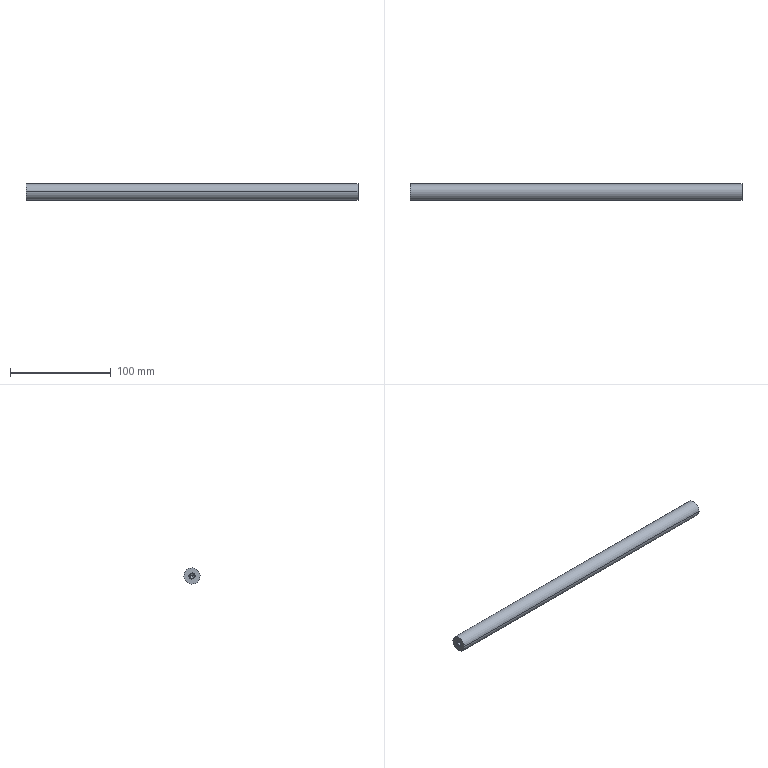Component | SolidWorks | DoubleFilmTransport-1_GuideRod-2 | 1 solid | 16 faces | box 330 x 16 x 16 mm | volume 65501 mm3 | cone 8 | cylinder 6 | plane 2 | commonest cylinder face diameters 5 x4 16 x2
build123d program:
from build123d import *


with BuildPart() as part:
    # Sketch1 → Revolve1 (revolve)
    with BuildSketch(Plane.XZ, mode=Mode.PRIVATE) as revolve1_sk:
        Polygon((2.5, 144), (0, 142.498), (0, -142.498), (2.5, -144), (2.5, -164.475), (3.025, -165), (8, -165), (8, 165), (3.025, 165), (2.5, 164.475), align=None)
    revolve(revolve1_sk.sketch.rotate(Axis((0, 0, 165), (0, 0, -1)), 180), axis=Axis((0, 0, 165), (0, 0, -1)))


solid = part.part

# Placed as in the assembly
solid = solid.moved(Location((-300.059, 45.373, 13.5), (0, 90, 0)))
STEP:
#1=COLOUR_RGB('',0.7922,0.8196,0.9333);
#2=FILL_AREA_STYLE_COLOUR('',#1);
#3=FILL_AREA_STYLE('',(#2));
#4=SURFACE_STYLE_FILL_AREA(#3);
#5=SURFACE_SIDE_STYLE('',(#4));
#6=SURFACE_STYLE_USAGE(.BOTH.,#5);
#7=PRESENTATION_STYLE_ASSIGNMENT((#6));
#8=CARTESIAN_POINT('',(-5.338,1.885,0.5242));
#9=VERTEX_POINT('',#8);
#10=CARTESIAN_POINT('',(-5.338,1.688,0.5388));
#11=VERTEX_POINT('',#10);
#12=CARTESIAN_POINT('',(-5.338,1.786,0.5315));
#13=DIRECTION('',(-1.,-0.,-0.));
#14=DIRECTION('',(0.,-0.9973,0.0739));
#15=AXIS2_PLACEMENT_3D('',#12,#13,#14);
#16=CIRCLE('',#15,0.09843);
#17=EDGE_CURVE('',#9,#11,#16,.T.);
#18=ORIENTED_EDGE('',*,*,#17,.T.);
#19=CARTESIAN_POINT('',(-5.317,1.668,0.5403));
#20=VERTEX_POINT('',#19);
#21=CARTESIAN_POINT('',(-5.317,1.668,0.5403));
#22=DIRECTION('',(0.7071,-0.7052,0.05225));
#23=VECTOR('',#22,39.37);
#24=LINE('',#21,#23);
#25=EDGE_CURVE('',#11,#20,#24,.T.);
#26=ORIENTED_EDGE('',*,*,#25,.T.);
#27=CARTESIAN_POINT('',(-5.317,1.905,0.5227));
#28=VERTEX_POINT('',#27);
#29=CARTESIAN_POINT('',(-5.317,1.786,0.5315));
#30=DIRECTION('',(-1.,-0.,-0.));
#31=DIRECTION('',(0.,-0.9973,0.0739));
#32=AXIS2_PLACEMENT_3D('',#29,#30,#31);
#33=CIRCLE('',#32,0.1191);
#34=EDGE_CURVE('',#28,#20,#33,.T.);
#35=ORIENTED_EDGE('',*,*,#34,.F.);
#36=CARTESIAN_POINT('',(-5.317,1.905,0.5227));
#37=DIRECTION('',(0.7071,0.7052,-0.05225));
#38=VECTOR('',#37,39.37);
#39=LINE('',#36,#38);
#40=EDGE_CURVE('',#9,#28,#39,.T.);
#41=ORIENTED_EDGE('',*,*,#40,.F.);
#42=EDGE_LOOP('',(#18,#26,#35,#41));
#43=FACE_OUTER_BOUND('',#42,.T.);
#44=CARTESIAN_POINT('',(-5.317,1.786,0.5315));
#45=DIRECTION('',(1.,0.,0.));
#46=DIRECTION('',(0.,0.9973,-0.0739));
#47=AXIS2_PLACEMENT_3D('',#44,#45,#46);
#48=CONICAL_SURFACE('',#47,0.1191,0.7854);
#49=ADVANCED_FACE('',(#43),#48,.F.);
#50=CARTESIAN_POINT('',(-5.317,1.472,0.5548));
#51=VERTEX_POINT('',#50);
#52=CARTESIAN_POINT('',(-5.317,2.1,0.5082));
#53=VERTEX_POINT('',#52);
#54=CARTESIAN_POINT('',(-5.317,1.786,0.5315));
#55=DIRECTION('',(-1.,-0.,-0.));
#56=DIRECTION('',(0.,-0.9973,0.0739));
#57=AXIS2_PLACEMENT_3D('',#54,#55,#56);
#58=CIRCLE('',#57,0.315);
#59=EDGE_CURVE('',#51,#53,#58,.T.);
#60=ORIENTED_EDGE('',*,*,#59,.T.);
#61=CARTESIAN_POINT('',(-18.309,2.1,0.5082));
#62=VERTEX_POINT('',#61);
#63=CARTESIAN_POINT('',(-5.317,2.1,0.5082));
#64=DIRECTION('',(-1.,-0.,-0.));
#65=VECTOR('',#64,39.37);
#66=LINE('',#63,#65);
#67=EDGE_CURVE('',#53,#62,#66,.T.);
#68=ORIENTED_EDGE('',*,*,#67,.T.);
#69=CARTESIAN_POINT('',(-18.309,1.472,0.5548));
#70=VERTEX_POINT('',#69);
#71=CARTESIAN_POINT('',(-18.309,1.786,0.5315));
#72=DIRECTION('',(-1.,-0.,-0.));
#73=DIRECTION('',(0.,-0.9973,0.0739));
#74=AXIS2_PLACEMENT_3D('',#71,#72,#73);
#75=CIRCLE('',#74,0.315);
#76=EDGE_CURVE('',#70,#62,#75,.T.);
#77=ORIENTED_EDGE('',*,*,#76,.F.);
#78=CARTESIAN_POINT('',(-5.317,1.472,0.5548));
#79=DIRECTION('',(-1.,-0.,-0.));
#80=VECTOR('',#79,39.37);
#81=LINE('',#78,#80);
#82=EDGE_CURVE('',#51,#70,#81,.T.);
#83=ORIENTED_EDGE('',*,*,#82,.F.);
#84=EDGE_LOOP('',(#60,#68,#77,#83));
#85=FACE_OUTER_BOUND('',#84,.T.);
#86=CARTESIAN_POINT('',(-5.317,1.786,0.5315));
#87=DIRECTION('',(-1.,-0.,-0.));
#88=DIRECTION('',(0.,-0.9973,0.0739));
#89=AXIS2_PLACEMENT_3D('',#86,#87,#88);
#90=CYLINDRICAL_SURFACE('',#89,0.315);
#91=ADVANCED_FACE('',(#85),#90,.T.);
#92=CARTESIAN_POINT('',(-18.289,1.885,0.5242));
#93=VERTEX_POINT('',#92);
#94=CARTESIAN_POINT('',(-18.289,1.688,0.5388));
#95=VERTEX_POINT('',#94);
#96=CARTESIAN_POINT('',(-18.289,1.786,0.5315));
#97=DIRECTION('',(-1.,-0.,-0.));
#98=DIRECTION('',(0.,-0.9973,0.0739));
#99=AXIS2_PLACEMENT_3D('',#96,#97,#98);
#100=CIRCLE('',#99,0.09843);
#101=EDGE_CURVE('',#93,#95,#100,.T.);
#102=ORIENTED_EDGE('',*,*,#101,.F.);
#103=CARTESIAN_POINT('',(-18.309,1.905,0.5227));
#104=VERTEX_POINT('',#103);
#105=CARTESIAN_POINT('',(-18.289,1.885,0.5242));
#106=DIRECTION('',(-0.7071,0.7052,-0.05225));
#107=VECTOR('',#106,39.37);
#108=LINE('',#105,#107);
#109=EDGE_CURVE('',#93,#104,#108,.T.);
#110=ORIENTED_EDGE('',*,*,#109,.T.);
#111=CARTESIAN_POINT('',(-18.309,1.668,0.5403));
#112=VERTEX_POINT('',#111);
#113=CARTESIAN_POINT('',(-18.309,1.786,0.5315));
#114=DIRECTION('',(-1.,-0.,-0.));
#115=DIRECTION('',(0.,-0.9973,0.0739));
#116=AXIS2_PLACEMENT_3D('',#113,#114,#115);
#117=CIRCLE('',#116,0.1191);
#118=EDGE_CURVE('',#104,#112,#117,.T.);
#119=ORIENTED_EDGE('',*,*,#118,.T.);
#120=CARTESIAN_POINT('',(-18.289,1.688,0.5388));
#121=DIRECTION('',(-0.7071,-0.7052,0.05225));
#122=VECTOR('',#121,39.37);
#123=LINE('',#120,#122);
#124=EDGE_CURVE('',#95,#112,#123,.T.);
#125=ORIENTED_EDGE('',*,*,#124,.F.);
#126=EDGE_LOOP('',(#102,#110,#119,#125));
#127=FACE_OUTER_BOUND('',#126,.T.);
#128=CARTESIAN_POINT('',(-18.289,1.786,0.5315));
#129=DIRECTION('',(-1.,-0.,-0.));
#130=DIRECTION('',(0.,-0.9973,0.0739));
#131=AXIS2_PLACEMENT_3D('',#128,#129,#130);
#132=CONICAL_SURFACE('',#131,0.09843,0.7854);
#133=ADVANCED_FACE('',(#127),#132,.F.);
#134=CARTESIAN_POINT('',(-17.483,1.885,0.5242));
#135=VERTEX_POINT('',#134);
#136=CARTESIAN_POINT('',(-17.483,1.688,0.5388));
#137=VERTEX_POINT('',#136);
#138=CARTESIAN_POINT('',(-17.483,1.786,0.5315));
#139=DIRECTION('',(-1.,-0.,-0.));
#140=DIRECTION('',(0.,-0.9973,0.0739));
#141=AXIS2_PLACEMENT_3D('',#138,#139,#140);
#142=CIRCLE('',#141,0.09843);
#143=EDGE_CURVE('',#135,#137,#142,.T.);
#144=ORIENTED_EDGE('',*,*,#143,.F.);
#145=CARTESIAN_POINT('',(-5.317,1.885,0.5242));
#146=DIRECTION('',(-1.,-0.,-0.));
#147=VECTOR('',#146,39.37);
#148=LINE('',#145,#147);
#149=EDGE_CURVE('',#135,#93,#148,.T.);
#150=ORIENTED_EDGE('',*,*,#149,.T.);
#151=ORIENTED_EDGE('',*,*,#101,.T.);
#152=CARTESIAN_POINT('',(-5.317,1.688,0.5388));
#153=DIRECTION('',(-1.,-0.,-0.));
#154=VECTOR('',#153,39.37);
#155=LINE('',#152,#154);
#156=EDGE_CURVE('',#137,#95,#155,.T.);
#157=ORIENTED_EDGE('',*,*,#156,.F.);
#158=EDGE_LOOP('',(#144,#150,#151,#157));
#159=FACE_OUTER_BOUND('',#158,.T.);
#160=CARTESIAN_POINT('',(-5.317,1.786,0.5315));
#161=DIRECTION('',(-1.,-0.,-0.));
#162=DIRECTION('',(0.,-0.9973,0.0739));
#163=AXIS2_PLACEMENT_3D('',#160,#161,#162);
#164=CYLINDRICAL_SURFACE('',#163,0.09843);
#165=ADVANCED_FACE('',(#159),#164,.F.);
#166=CARTESIAN_POINT('',(-17.424,1.786,0.5315));
#167=VERTEX_POINT('',#166);
#168=CARTESIAN_POINT('',(-17.424,1.786,0.5315));
#169=DIRECTION('',(-0.515,-0.8548,0.06334));
#170=VECTOR('',#169,39.37);
#171=LINE('',#168,#170);
#172=EDGE_CURVE('',#167,#137,#171,.T.);
#173=ORIENTED_EDGE('',*,*,#172,.F.);
#174=CARTESIAN_POINT('',(-17.424,1.786,0.5315));
#175=DIRECTION('',(-0.515,0.8548,-0.06334));
#176=VECTOR('',#175,39.37);
#177=LINE('',#174,#176);
#178=EDGE_CURVE('',#167,#135,#177,.T.);
#179=ORIENTED_EDGE('',*,*,#178,.T.);
#180=ORIENTED_EDGE('',*,*,#143,.T.);
#181=EDGE_LOOP('',(#173,#179,#180));
#182=FACE_OUTER_BOUND('',#181,.T.);
#183=CARTESIAN_POINT('',(-56.794,1.786,0.5315));
#184=DIRECTION('',(-1.,-0.,-0.));
#185=DIRECTION('',(0.,-0.9973,0.0739));
#186=AXIS2_PLACEMENT_3D('',#183,#184,#185);
#187=CONICAL_SURFACE('',#186,65.523,1.03);
#188=ADVANCED_FACE('',(#182),#187,.F.);
#189=CARTESIAN_POINT('',(-6.203,1.786,0.5315));
#190=VERTEX_POINT('',#189);
#191=CARTESIAN_POINT('',(-6.144,1.885,0.5242));
#192=VERTEX_POINT('',#191);
#193=CARTESIAN_POINT('',(-6.144,1.885,0.5242));
#194=DIRECTION('',(0.515,0.8548,-0.06334));
#195=VECTOR('',#194,39.37);
#196=LINE('',#193,#195);
#197=EDGE_CURVE('',#190,#192,#196,.T.);
#198=ORIENTED_EDGE('',*,*,#197,.F.);
#199=CARTESIAN_POINT('',(-6.144,1.688,0.5388));
#200=VERTEX_POINT('',#199);
#201=CARTESIAN_POINT('',(-6.144,1.688,0.5388));
#202=DIRECTION('',(0.515,-0.8548,0.06334));
#203=VECTOR('',#202,39.37);
#204=LINE('',#201,#203);
#205=EDGE_CURVE('',#190,#200,#204,.T.);
#206=ORIENTED_EDGE('',*,*,#205,.T.);
#207=CARTESIAN_POINT('',(-6.144,1.786,0.5315));
#208=DIRECTION('',(-1.,-0.,-0.));
#209=DIRECTION('',(0.,-0.9973,0.0739));
#210=AXIS2_PLACEMENT_3D('',#207,#208,#209);
#211=CIRCLE('',#210,0.09843);
#212=EDGE_CURVE('',#192,#200,#211,.T.);
#213=ORIENTED_EDGE('',*,*,#212,.F.);
#214=EDGE_LOOP('',(#198,#206,#213));
#215=FACE_OUTER_BOUND('',#214,.T.);
#216=CARTESIAN_POINT('',(-6.144,1.786,0.5315));
#217=DIRECTION('',(1.,0.,0.));
#218=DIRECTION('',(0.,0.9973,-0.0739));
#219=AXIS2_PLACEMENT_3D('',#216,#217,#218);
#220=CONICAL_SURFACE('',#219,0.09843,1.03);
#221=ADVANCED_FACE('',(#215),#220,.F.);
#222=ORIENTED_EDGE('',*,*,#17,.F.);
#223=CARTESIAN_POINT('',(-5.317,1.885,0.5242));
#224=DIRECTION('',(-1.,-0.,-0.));
#225=VECTOR('',#224,39.37);
#226=LINE('',#223,#225);
#227=EDGE_CURVE('',#9,#192,#226,.T.);
#228=ORIENTED_EDGE('',*,*,#227,.T.);
#229=ORIENTED_EDGE('',*,*,#212,.T.);
#230=CARTESIAN_POINT('',(-5.317,1.688,0.5388));
#231=DIRECTION('',(-1.,-0.,-0.));
#232=VECTOR('',#231,39.37);
#233=LINE('',#230,#232);
#234=EDGE_CURVE('',#11,#200,#233,.T.);
#235=ORIENTED_EDGE('',*,*,#234,.F.);
#236=EDGE_LOOP('',(#222,#228,#229,#235));
#237=FACE_OUTER_BOUND('',#236,.T.);
#238=CARTESIAN_POINT('',(-5.317,1.786,0.5315));
#239=DIRECTION('',(-1.,-0.,-0.));
#240=DIRECTION('',(0.,-0.9973,0.0739));
#241=AXIS2_PLACEMENT_3D('',#238,#239,#240);
#242=CYLINDRICAL_SURFACE('',#241,0.09843);
#243=ADVANCED_FACE('',(#237),#242,.F.);
#244=ORIENTED_EDGE('',*,*,#227,.F.);
#245=CARTESIAN_POINT('',(-5.338,1.786,0.5315));
#246=DIRECTION('',(-1.,-0.,-0.));
#247=DIRECTION('',(0.,-0.9973,0.0739));
#248=AXIS2_PLACEMENT_3D('',#245,#246,#247);
#249=CIRCLE('',#248,0.09843);
#250=EDGE_CURVE('',#11,#9,#249,.T.);
#251=ORIENTED_EDGE('',*,*,#250,.F.);
#252=ORIENTED_EDGE('',*,*,#234,.T.);
#253=CARTESIAN_POINT('',(-6.144,1.786,0.5315));
#254=DIRECTION('',(-1.,-0.,-0.));
#255=DIRECTION('',(0.,-0.9973,0.0739));
#256=AXIS2_PLACEMENT_3D('',#253,#254,#255);
#257=CIRCLE('',#256,0.09843);
#258=EDGE_CURVE('',#200,#192,#257,.T.);
#259=ORIENTED_EDGE('',*,*,#258,.T.);
#260=EDGE_LOOP('',(#244,#251,#252,#259));
#261=FACE_OUTER_BOUND('',#260,.T.);
#262=CARTESIAN_POINT('',(-5.317,1.786,0.5315));
#263=DIRECTION('',(-1.,-0.,-0.));
#264=DIRECTION('',(0.,-0.9973,0.0739));
#265=AXIS2_PLACEMENT_3D('',#262,#263,#264);
#266=CYLINDRICAL_SURFACE('',#265,0.09843);
#267=ADVANCED_FACE('',(#261),#266,.F.);
#268=ORIENTED_EDGE('',*,*,#205,.F.);
#269=ORIENTED_EDGE('',*,*,#197,.T.);
#270=ORIENTED_EDGE('',*,*,#258,.F.);
#271=EDGE_LOOP('',(#268,#269,#270));
#272=FACE_OUTER_BOUND('',#271,.T.);
#273=CARTESIAN_POINT('',(-6.144,1.786,0.5315));
#274=DIRECTION('',(1.,0.,0.));
#275=DIRECTION('',(0.,0.9973,-0.0739));
#276=AXIS2_PLACEMENT_3D('',#273,#274,#275);
#277=CONICAL_SURFACE('',#276,0.09843,1.03);
#278=ADVANCED_FACE('',(#272),#277,.F.);
#279=ORIENTED_EDGE('',*,*,#178,.F.);
#280=ORIENTED_EDGE('',*,*,#172,.T.);
#281=CARTESIAN_POINT('',(-17.483,1.786,0.5315));
#282=DIRECTION('',(-1.,-0.,-0.));
#283=DIRECTION('',(0.,-0.9973,0.0739));
#284=AXIS2_PLACEMENT_3D('',#281,#282,#283);
#285=CIRCLE('',#284,0.09843);
#286=EDGE_CURVE('',#137,#135,#285,.T.);
#287=ORIENTED_EDGE('',*,*,#286,.T.);
#288=EDGE_LOOP('',(#279,#280,#287));
#289=FACE_OUTER_BOUND('',#288,.T.);
#290=CARTESIAN_POINT('',(-56.794,1.786,0.5315));
#291=DIRECTION('',(-1.,-0.,-0.));
#292=DIRECTION('',(0.,-0.9973,0.0739));
#293=AXIS2_PLACEMENT_3D('',#290,#291,#292);
#294=CONICAL_SURFACE('',#293,65.523,1.03);
#295=ADVANCED_FACE('',(#289),#294,.F.);
#296=ORIENTED_EDGE('',*,*,#149,.F.);
#297=ORIENTED_EDGE('',*,*,#286,.F.);
#298=ORIENTED_EDGE('',*,*,#156,.T.);
#299=CARTESIAN_POINT('',(-18.289,1.786,0.5315));
#300=DIRECTION('',(-1.,-0.,-0.));
#301=DIRECTION('',(0.,-0.9973,0.0739));
#302=AXIS2_PLACEMENT_3D('',#299,#300,#301);
#303=CIRCLE('',#302,0.09843);
#304=EDGE_CURVE('',#95,#93,#303,.T.);
#305=ORIENTED_EDGE('',*,*,#304,.T.);
#306=EDGE_LOOP('',(#296,#297,#298,#305));
#307=FACE_OUTER_BOUND('',#306,.T.);
#308=CARTESIAN_POINT('',(-5.317,1.786,0.5315));
#309=DIRECTION('',(-1.,-0.,-0.));
#310=DIRECTION('',(0.,-0.9973,0.0739));
#311=AXIS2_PLACEMENT_3D('',#308,#309,#310);
#312=CYLINDRICAL_SURFACE('',#311,0.09843);
#313=ADVANCED_FACE('',(#307),#312,.F.);
#314=ORIENTED_EDGE('',*,*,#109,.F.);
#315=ORIENTED_EDGE('',*,*,#304,.F.);
#316=ORIENTED_EDGE('',*,*,#124,.T.);
#317=CARTESIAN_POINT('',(-18.309,1.786,0.5315));
#318=DIRECTION('',(-1.,-0.,-0.));
#319=DIRECTION('',(0.,-0.9973,0.0739));
#320=AXIS2_PLACEMENT_3D('',#317,#318,#319);
#321=CIRCLE('',#320,0.1191);
#322=EDGE_CURVE('',#112,#104,#321,.T.);
#323=ORIENTED_EDGE('',*,*,#322,.T.);
#324=EDGE_LOOP('',(#314,#315,#316,#323));
#325=FACE_OUTER_BOUND('',#324,.T.);
#326=CARTESIAN_POINT('',(-18.289,1.786,0.5315));
#327=DIRECTION('',(-1.,-0.,-0.));
#328=DIRECTION('',(0.,-0.9973,0.0739));
#329=AXIS2_PLACEMENT_3D('',#326,#327,#328);
#330=CONICAL_SURFACE('',#329,0.09843,0.7854);
#331=ADVANCED_FACE('',(#325),#330,.F.);
#332=ORIENTED_EDGE('',*,*,#76,.T.);
#333=CARTESIAN_POINT('',(-18.309,1.786,0.5315));
#334=DIRECTION('',(-1.,-0.,-0.));
#335=DIRECTION('',(0.,-0.9973,0.0739));
#336=AXIS2_PLACEMENT_3D('',#333,#334,#335);
#337=CIRCLE('',#336,0.315);
#338=EDGE_CURVE('',#62,#70,#337,.T.);
#339=ORIENTED_EDGE('',*,*,#338,.T.);
#340=EDGE_LOOP('',(#332,#339));
#341=FACE_OUTER_BOUND('',#340,.T.);
#342=ORIENTED_EDGE('',*,*,#322,.F.);
#343=ORIENTED_EDGE('',*,*,#118,.F.);
#344=EDGE_LOOP('',(#342,#343));
#345=FACE_BOUND('',#344,.T.);
#346=CARTESIAN_POINT('',(-18.309,1.905,0.5227));
#347=DIRECTION('',(-1.,-0.,-0.));
#348=DIRECTION('',(0.,-0.9973,0.0739));
#349=AXIS2_PLACEMENT_3D('',#346,#347,#348);
#350=PLANE('',#349);
#351=ADVANCED_FACE('',(#341,#345),#350,.T.);
#352=ORIENTED_EDGE('',*,*,#67,.F.);
#353=CARTESIAN_POINT('',(-5.317,1.786,0.5315));
#354=DIRECTION('',(-1.,-0.,-0.));
#355=DIRECTION('',(0.,-0.9973,0.0739));
#356=AXIS2_PLACEMENT_3D('',#353,#354,#355);
#357=CIRCLE('',#356,0.315);
#358=EDGE_CURVE('',#53,#51,#357,.T.);
#359=ORIENTED_EDGE('',*,*,#358,.T.);
#360=ORIENTED_EDGE('',*,*,#82,.T.);
#361=ORIENTED_EDGE('',*,*,#338,.F.);
#362=EDGE_LOOP('',(#352,#359,#360,#361));
#363=FACE_OUTER_BOUND('',#362,.T.);
#364=CARTESIAN_POINT('',(-5.317,1.786,0.5315));
#365=DIRECTION('',(-1.,-0.,-0.));
#366=DIRECTION('',(0.,-0.9973,0.0739));
#367=AXIS2_PLACEMENT_3D('',#364,#365,#366);
#368=CYLINDRICAL_SURFACE('',#367,0.315);
#369=ADVANCED_FACE('',(#363),#368,.T.);
#370=ORIENTED_EDGE('',*,*,#34,.T.);
#371=CARTESIAN_POINT('',(-5.317,1.786,0.5315));
#372=DIRECTION('',(-1.,-0.,-0.));
#373=DIRECTION('',(0.,-0.9973,0.0739));
#374=AXIS2_PLACEMENT_3D('',#371,#372,#373);
#375=CIRCLE('',#374,0.1191);
#376=EDGE_CURVE('',#20,#28,#375,.T.);
#377=ORIENTED_EDGE('',*,*,#376,.T.);
#378=EDGE_LOOP('',(#370,#377));
#379=FACE_BOUND('',#378,.T.);
#380=ORIENTED_EDGE('',*,*,#59,.F.);
#381=ORIENTED_EDGE('',*,*,#358,.F.);
#382=EDGE_LOOP('',(#380,#381));
#383=FACE_OUTER_BOUND('',#382,.T.);
#384=CARTESIAN_POINT('',(-5.317,2.1,0.5082));
#385=DIRECTION('',(1.,0.,0.));
#386=DIRECTION('',(-0.,0.9973,-0.0739));
#387=AXIS2_PLACEMENT_3D('',#384,#385,#386);
#388=PLANE('',#387);
#389=ADVANCED_FACE('',(#379,#383),#388,.T.);
#390=ORIENTED_EDGE('',*,*,#25,.F.);
#391=ORIENTED_EDGE('',*,*,#250,.T.);
#392=ORIENTED_EDGE('',*,*,#40,.T.);
#393=ORIENTED_EDGE('',*,*,#376,.F.);
#394=EDGE_LOOP('',(#390,#391,#392,#393));
#395=FACE_OUTER_BOUND('',#394,.T.);
#396=CARTESIAN_POINT('',(-5.317,1.786,0.5315));
#397=DIRECTION('',(1.,0.,0.));
#398=DIRECTION('',(0.,0.9973,-0.0739));
#399=AXIS2_PLACEMENT_3D('',#396,#397,#398);
#400=CONICAL_SURFACE('',#399,0.1191,0.7854);
#401=ADVANCED_FACE('',(#395),#400,.F.);
#402=CLOSED_SHELL('',(#49,#91,#133,#165,#188,#221,#243,#267,#278,#295,#313,#331,#351,#369,#389,#401));
#403=MANIFOLD_SOLID_BREP('',#402);
#404=STYLED_ITEM('',(#7),#403);
#405=(LENGTH_UNIT()NAMED_UNIT(*)SI_UNIT($,.METRE.));
#406=LENGTH_MEASURE_WITH_UNIT(LENGTH_MEASURE(0.0254),#405);
#407=DIMENSIONAL_EXPONENTS(1.,0.,0.,0.,0.,0.,0.);
#408=(CONVERSION_BASED_UNIT('',#406)LENGTH_UNIT()NAMED_UNIT(#407));
#409=UNCERTAINTY_MEASURE_WITH_UNIT(LENGTH_MEASURE(0.00001),#408,'','');
#410=(NAMED_UNIT(*)PLANE_ANGLE_UNIT()SI_UNIT($,.RADIAN.));
#411=(NAMED_UNIT(*)SI_UNIT($,.STERADIAN.)SOLID_ANGLE_UNIT());
#412=(GEOMETRIC_REPRESENTATION_CONTEXT(3)GLOBAL_UNCERTAINTY_ASSIGNED_CONTEXT((#409))GLOBAL_UNIT_ASSIGNED_CONTEXT((#408,#410,#411))REPRESENTATION_CONTEXT('',''));
#413=MECHANICAL_DESIGN_GEOMETRIC_PRESENTATION_REPRESENTATION('',(#404),#412);
#414=CARTESIAN_POINT('',(0.,0.,0.));
#415=DIRECTION('',(0.,0.,1.));
#416=DIRECTION('',(1.,0.,0.));
#417=AXIS2_PLACEMENT_3D('',#414,#415,#416);
#418=(LENGTH_UNIT()NAMED_UNIT(*)SI_UNIT($,.METRE.));
#419=LENGTH_MEASURE_WITH_UNIT(LENGTH_MEASURE(0.0254),#418);
#420=DIMENSIONAL_EXPONENTS(1.,0.,0.,0.,0.,0.,0.);
#421=(CONVERSION_BASED_UNIT('',#419)LENGTH_UNIT()NAMED_UNIT(#420));
#422=UNCERTAINTY_MEASURE_WITH_UNIT(LENGTH_MEASURE(0.00001),#421,'','');
#423=(NAMED_UNIT(*)PLANE_ANGLE_UNIT()SI_UNIT($,.RADIAN.));
#424=(NAMED_UNIT(*)SI_UNIT($,.STERADIAN.)SOLID_ANGLE_UNIT());
#425=(GEOMETRIC_REPRESENTATION_CONTEXT(3)GLOBAL_UNCERTAINTY_ASSIGNED_CONTEXT((#422))GLOBAL_UNIT_ASSIGNED_CONTEXT((#421,#423,#424))REPRESENTATION_CONTEXT('',''));
#426=ADVANCED_BREP_SHAPE_REPRESENTATION('',(#403,#417),#425);
#427=PRESENTATION_LAYER_ASSIGNMENT('','',(#404));